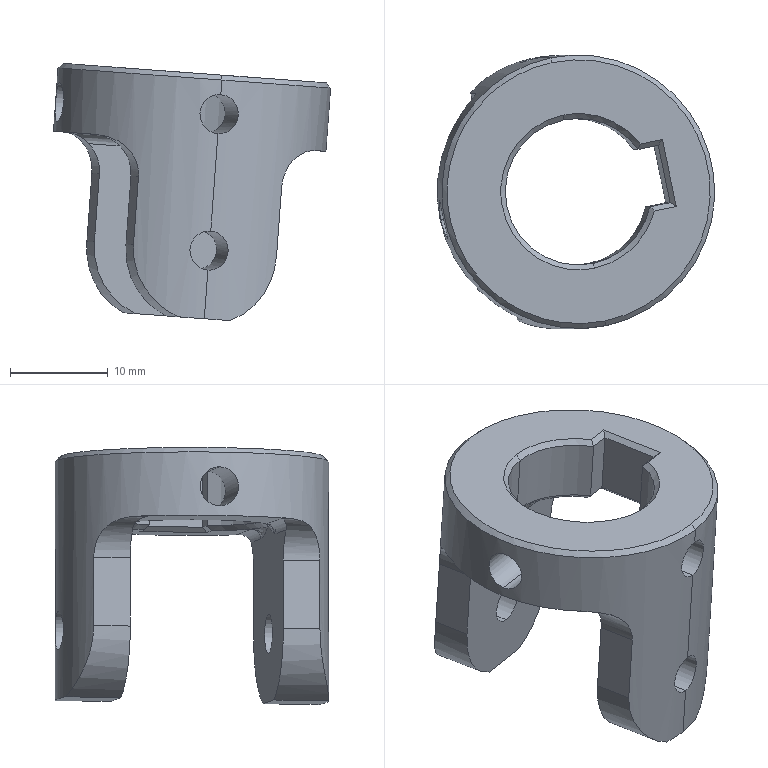Component | SolidWorks | DoubleFilmTransport-1_UniversalJointB-2 | 1 solid | 57 faces | volume 5409 mm3 | cylinder 25 | plane 20 | cone 8 | spline 4 | commonest cylinder face diameters 4 x8 15 x7 7.978 x4 2 x4 28 x2